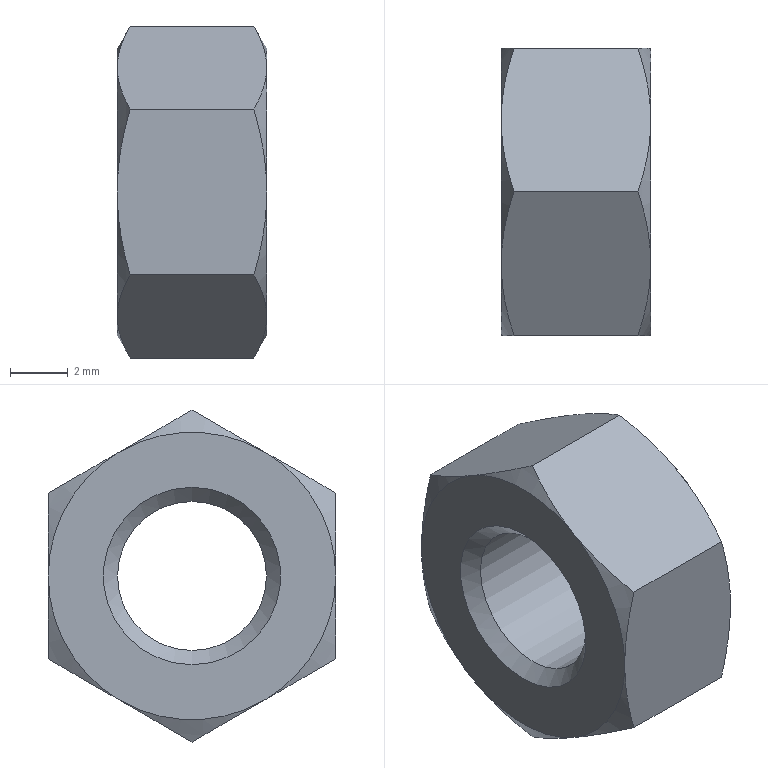Component | NX | GB-T6170_F-2000_M6X1_2 | 1 solid | 23 faces | volume 334 mm3 | cone 14 | plane 8 | cylinder 1 | commonest cylinder face diameters 5.188 x1